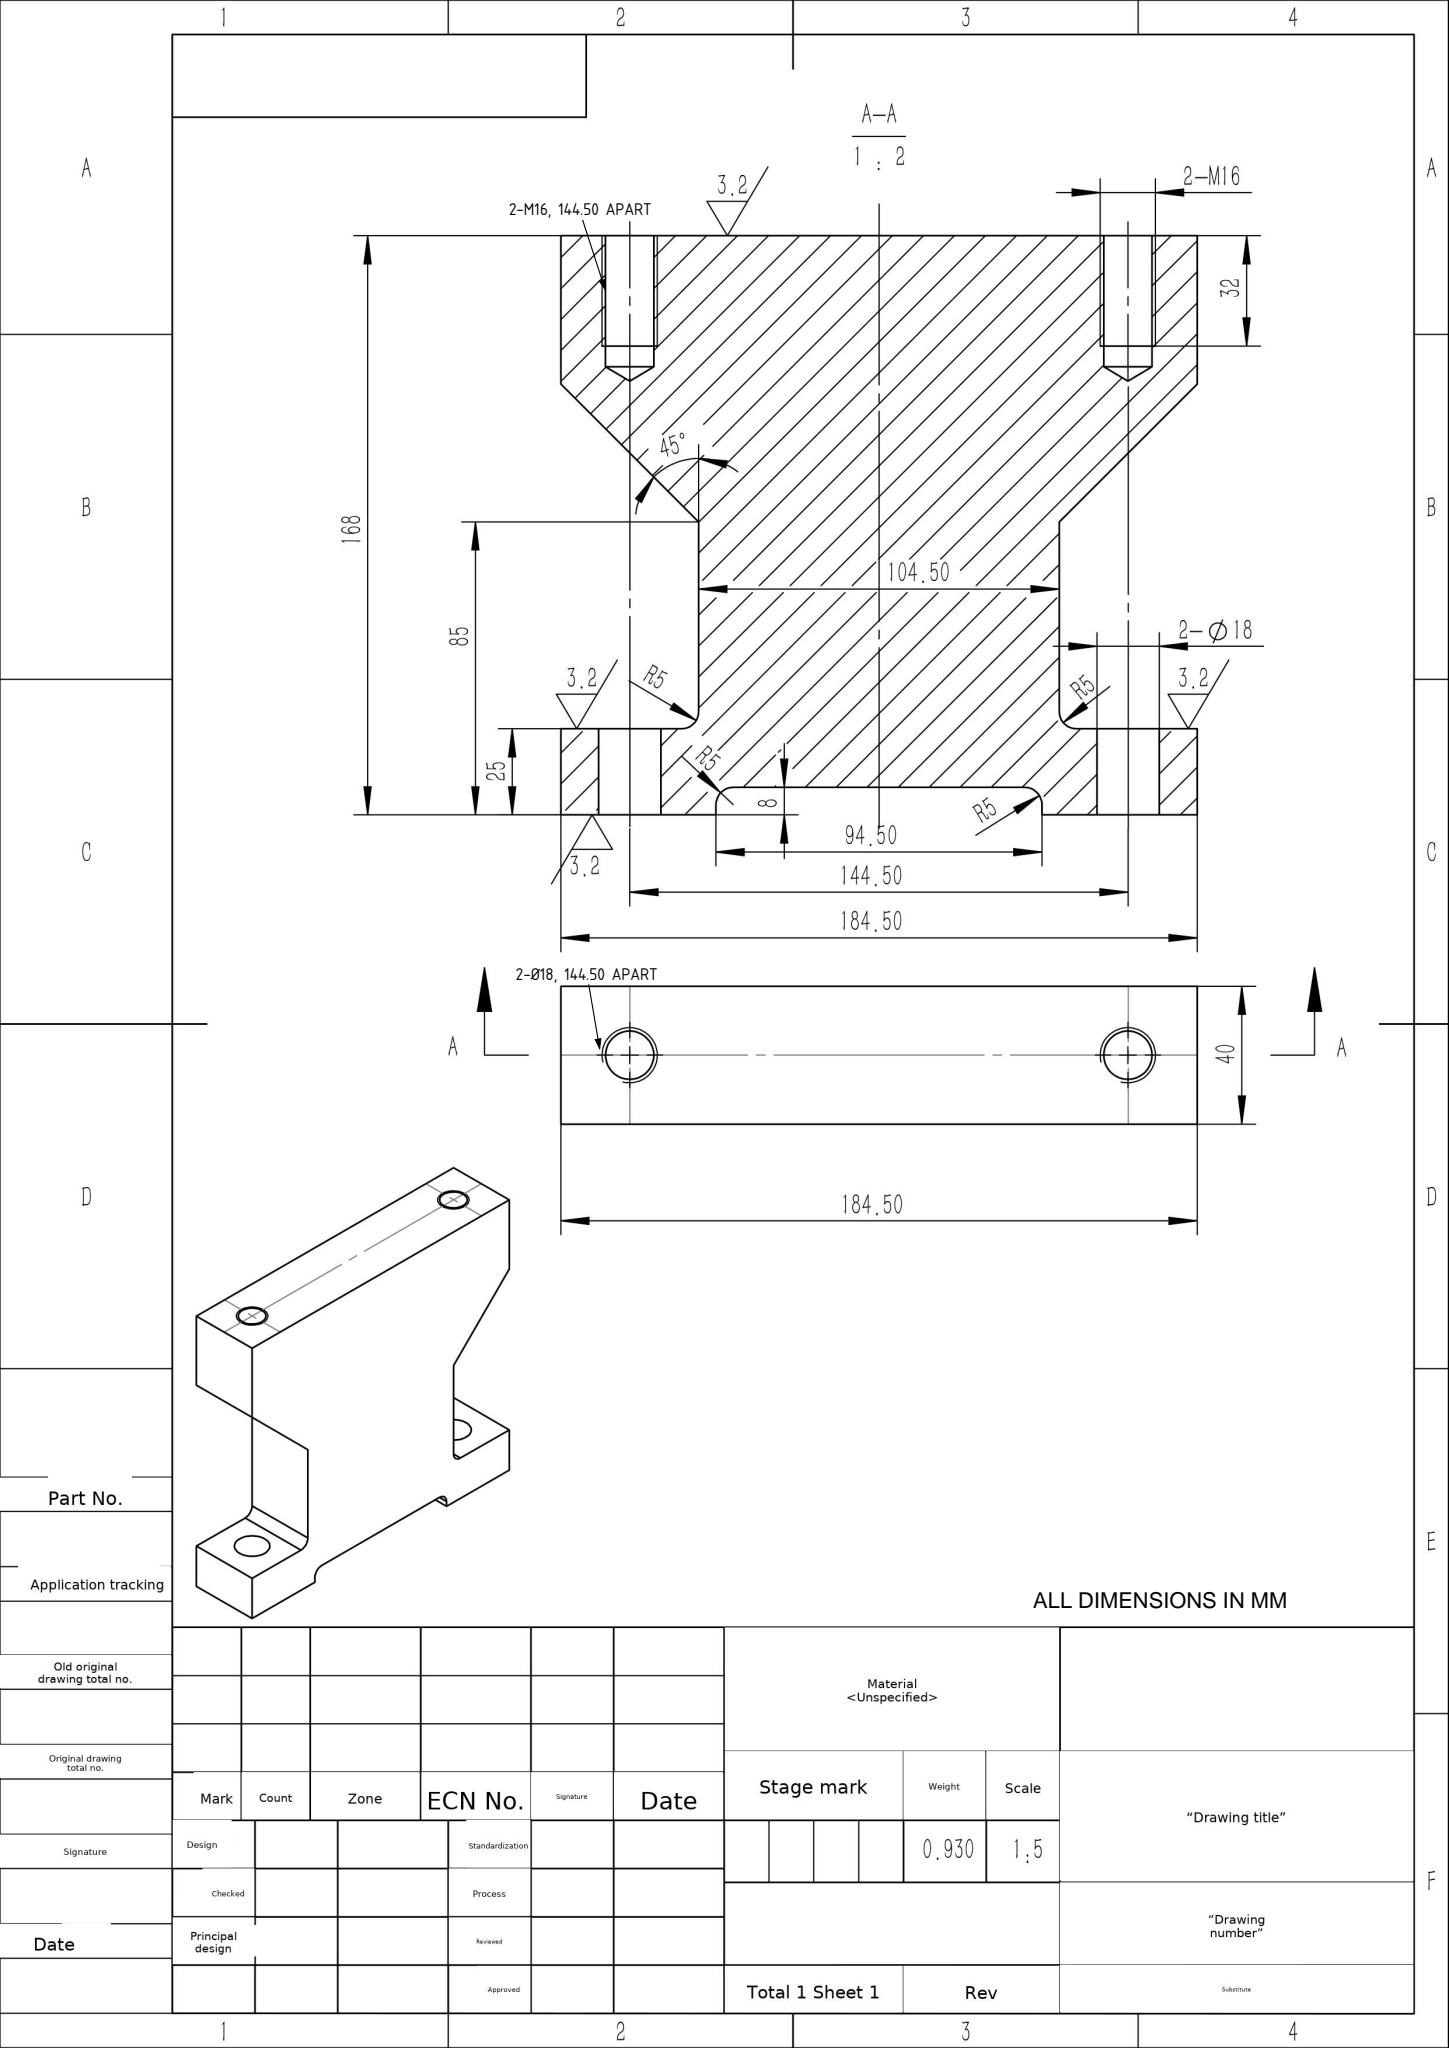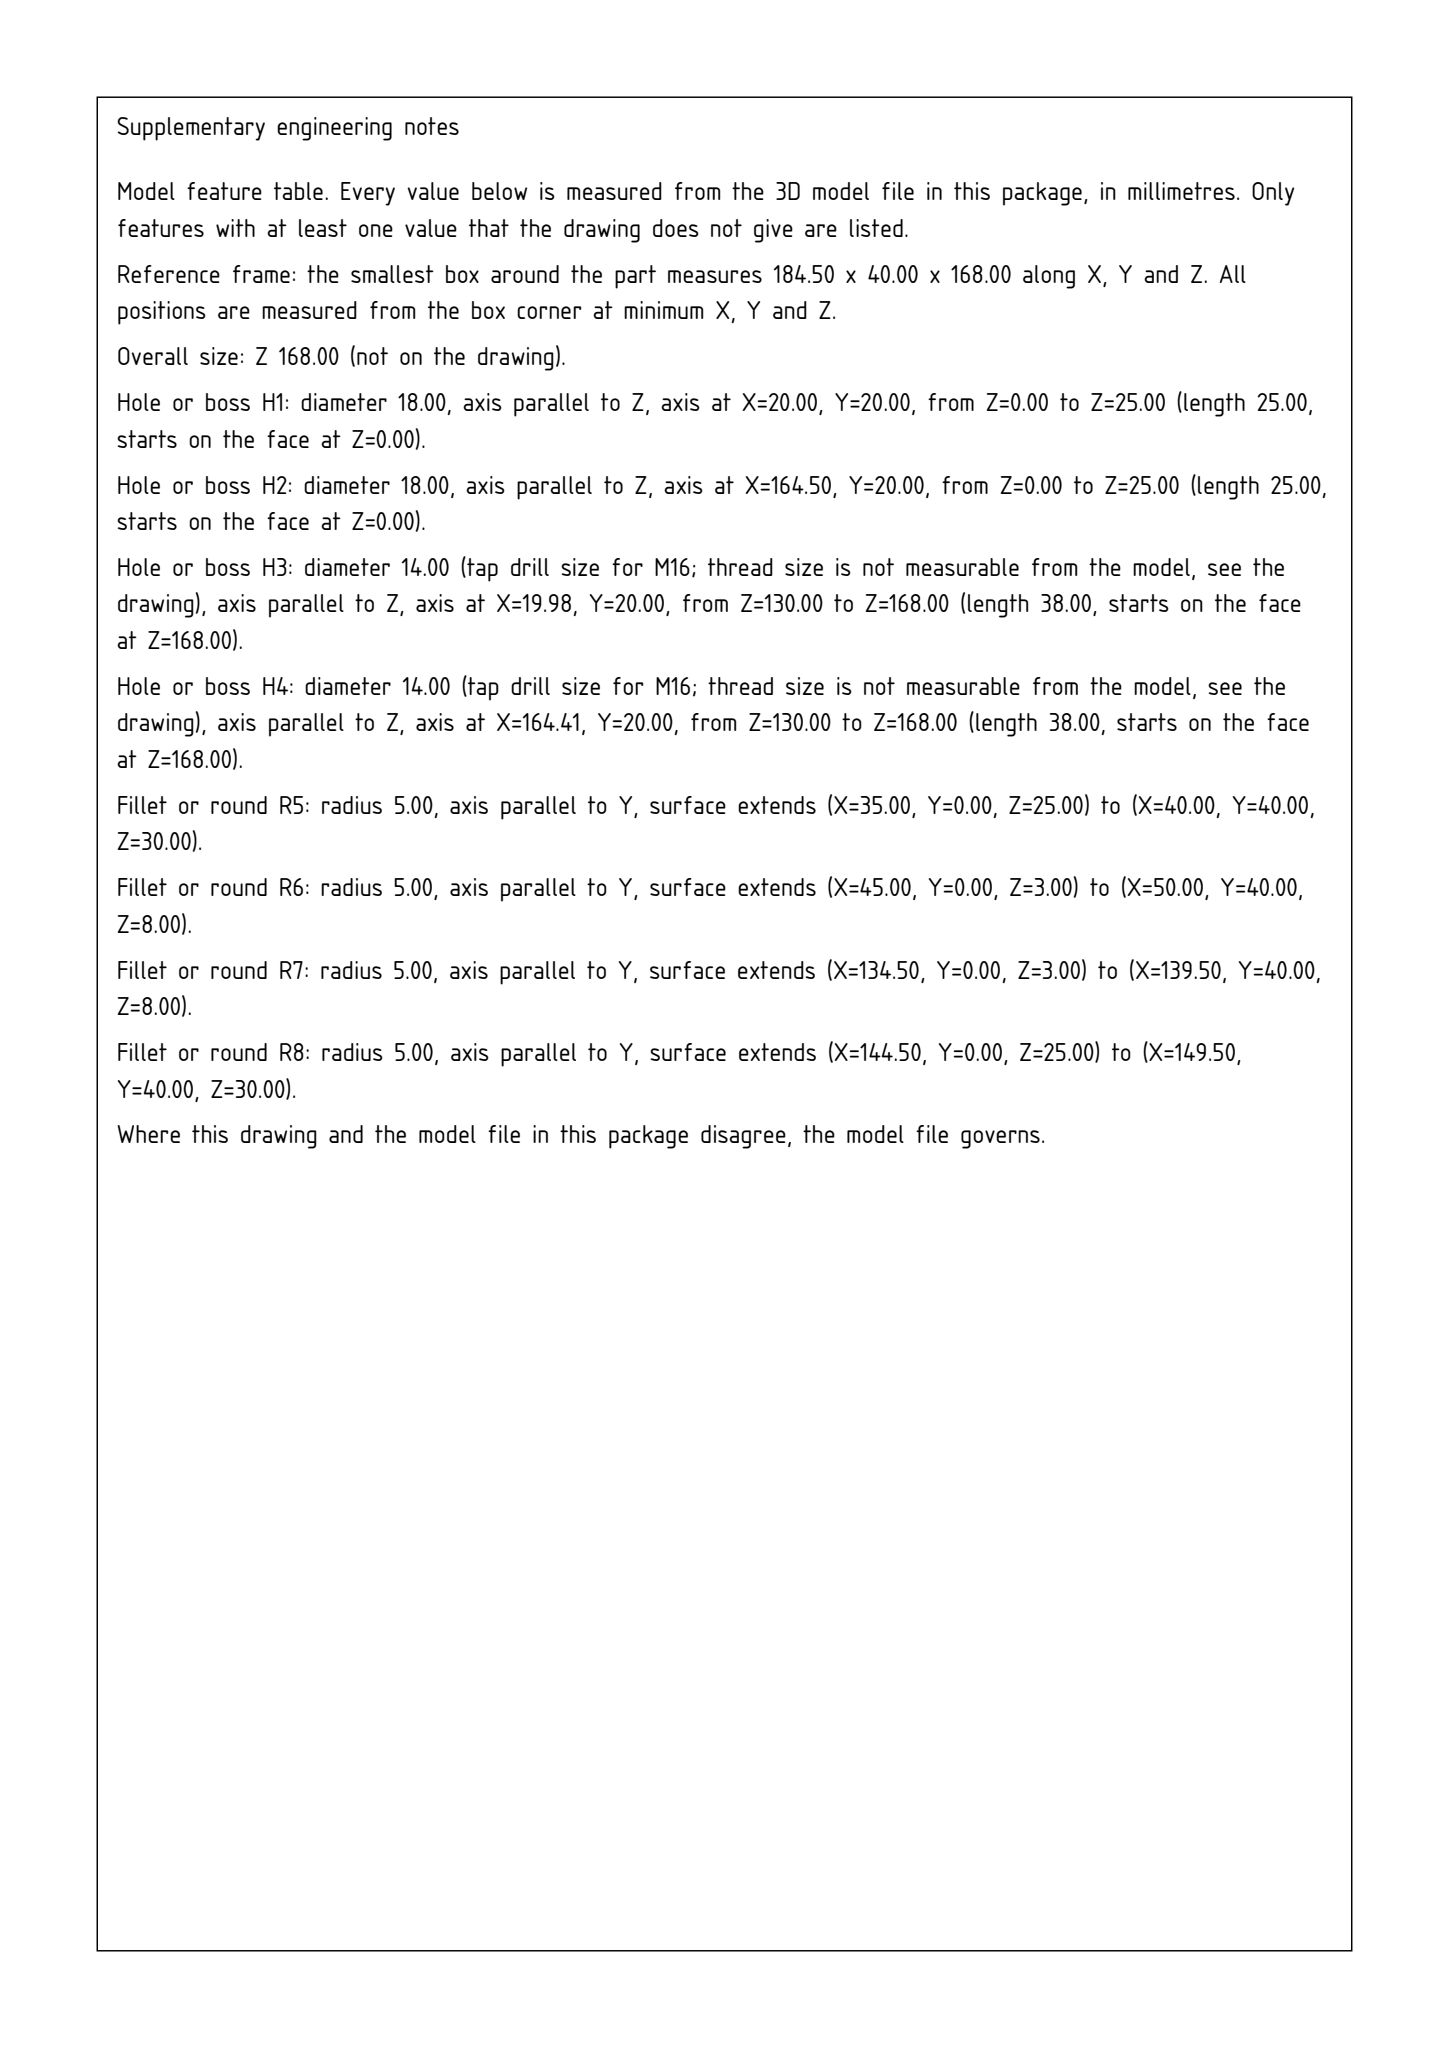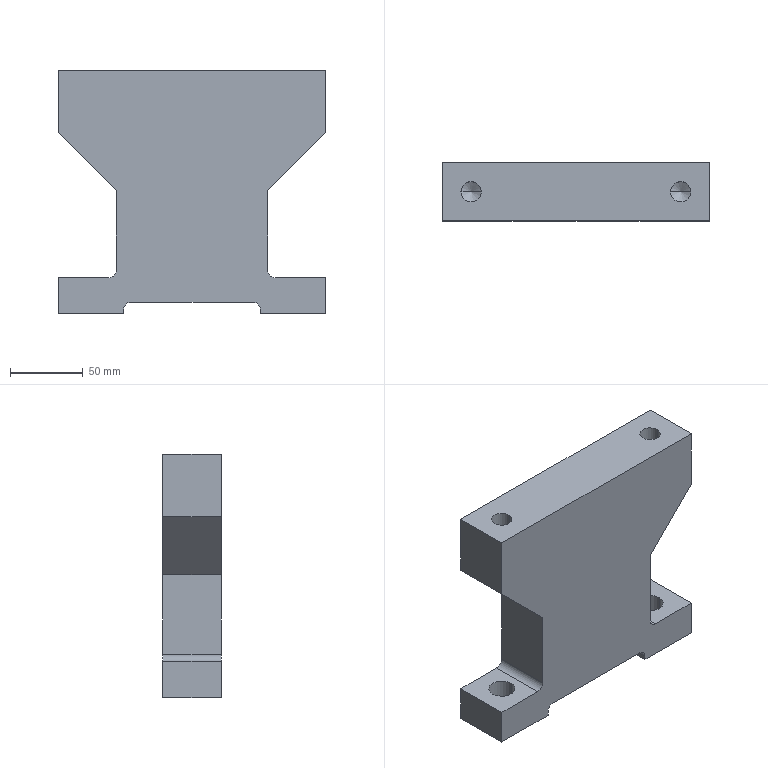Part | SolidWorks | mm | 1 solid | 34 faces | box 184.5 x 40 x 168 mm | volume 929604 mm3 | plane 18 | cylinder 12 | cone 4 | commonest cylinder face diameters 14 x4 18 x4 10 x4
Drawing notes:
2-M16 AXES 20 FROM EACH END, 144.50 APART (SEE A-A) | from the solid: M16 bore dia 14 axes at x=20.0 and x=164.4; bbox x=184.5; spacing 144.5
2-Ø18 AXES 20 FROM EACH END, 144.50 APART, ON 40 WIDTH CL | from the solid: Ø18 holes axes at x=20.0 and x=164.5, y=20.0 (of 40); bbox x=184.5
build123d program:
from build123d import *

# Parameters (mm, degrees)
SKETCH1_W              = 184.5
SKETCH1_H              = 40
BOSS_EXTRUDE1_DEPTH    = 168
SKETCH2_W              = 94.5
SKETCH2_H              = 8
CUT_EXTRUDE1_DEPTH     = 253.714
CUT_EXTRUDE2_REACH     = 254.714
SKETCH3_R              = 9
FILLET1_R              = 5
M16_TAPPED_HOLE1_D     = 14
M16_TAPPED_HOLE1_DEPTH = 38
M16_TAPPED_HOLE1_TIP   = 4.206


with BuildPart() as part:
    # Sketch1 → Boss-Extrude1 (new body)
    with BuildSketch(Plane.XY):
        with Locations((92.25, 20)):
            Rectangle(SKETCH1_W, SKETCH1_H)
    extrude(amount=BOSS_EXTRUDE1_DEPTH)

    # Sketch2 → Cut-Extrude1 (cut, through all)
    with BuildSketch(Plane(origin=(0, 40, 0), x_dir=(1, 0, 0), z_dir=(0, 1, 0))):
        Polygon((184.5, -25), (144.5, -25), (144.5, -85), (184.5, -125), align=None)
        Polygon((0, -25), (40, -25), (40, -85), (0, -125), align=None)
        with Locations((92.25, -4)):
            Rectangle(SKETCH2_W, SKETCH2_H)
    extrude(amount=-CUT_EXTRUDE1_DEPTH, mode=Mode.SUBTRACT)

    # Sketch3 → Cut-Extrude2 (cut, up to next)
    with BuildSketch(Plane(origin=(0, 0, 0), x_dir=(-1, 0, 0), z_dir=(0, 0, -1)), mode=Mode.PRIVATE) as cut_extrude2_sk1:
        with Locations((-20, 20)):
            Circle(SKETCH3_R)
    cut_extrude2_tool1 = extrude(cut_extrude2_sk1.sketch, amount=-CUT_EXTRUDE2_REACH, mode=Mode.PRIVATE) & part.part
    # Sketch3 → Cut-Extrude2 (cut, up to next)
    with BuildSketch(Plane(origin=(0, 0, 0), x_dir=(-1, 0, 0), z_dir=(0, 0, -1)), mode=Mode.PRIVATE) as cut_extrude2_sk2:
        with Locations((-164.5, 20)):
            Circle(SKETCH3_R)
    cut_extrude2_tool2 = extrude(cut_extrude2_sk2.sketch, amount=-CUT_EXTRUDE2_REACH, mode=Mode.PRIVATE) & part.part
    add(cut_extrude2_tool1.solids().sort_by_distance((20, 20, 0))[0], mode=Mode.SUBTRACT)
    add(cut_extrude2_tool2.solids().sort_by_distance((164.5, 20, 0))[0], mode=Mode.SUBTRACT)

    # Fillet1
    fillet1_edges = [part.edges().sort_by_distance(p)[0] for p in [
        (144.5, 20, 25),
        (40, 20, 25),
        (45, 20, 8),
        (139.5, 20, 8),
    ]]
    fillet(fillet1_edges, radius=FILLET1_R)

    # M16 Tapped Hole1
    with Locations(Plane(origin=(164.413, 20, 168), x_dir=(1, 0, 0), z_dir=(0, 0, 1))):
        with Locations((0, 0), (-144.437, 0)):
            Hole(M16_TAPPED_HOLE1_D / 2, depth=M16_TAPPED_HOLE1_DEPTH)
            with Locations((0, 0, -(M16_TAPPED_HOLE1_DEPTH + M16_TAPPED_HOLE1_TIP / 2))):  # 118° drill point
                Cone(0, M16_TAPPED_HOLE1_D / 2, M16_TAPPED_HOLE1_TIP, mode=Mode.SUBTRACT)


solid = part.part